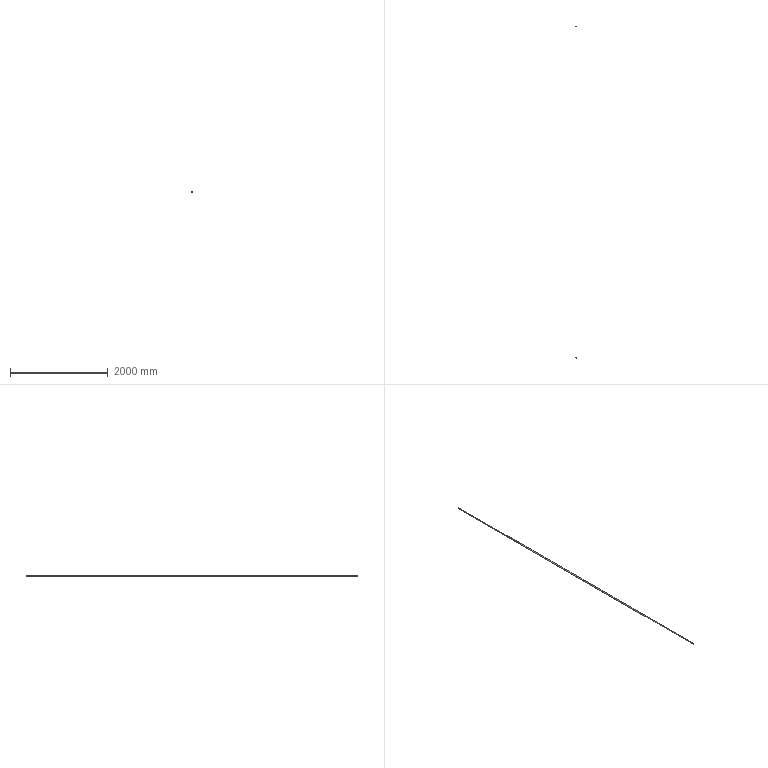Component | NX | 44_5_2 | 1 solid | 4 faces | volume 768383 mm3 | cylinder 2 | plane 2 | commonest cylinder face diameters 20 x1 16 x1